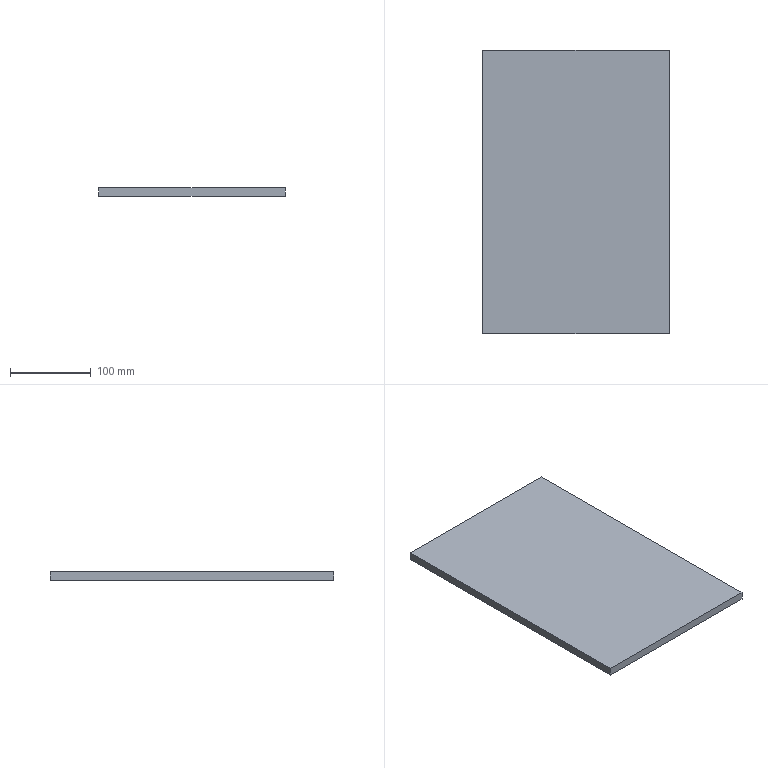Component | SolidWorks | ElectricalCabinetPanel-2 | 1 solid | 6 faces | box 230 x 350 x 10 mm | volume 805000 mm3 | plane 6
build123d program:
from build123d import *

# Parameters (mm, degrees)
SKETCH1_W           = 350
SKETCH1_H           = 230
BOSS_EXTRUDE1_DEPTH = 10


with BuildPart() as part:
    # Sketch1 → Boss-Extrude1 (new body)
    with BuildSketch(Plane.XY):
        with Locations((-175, -115)):
            Rectangle(SKETCH1_W, SKETCH1_H)
    extrude(amount=BOSS_EXTRUDE1_DEPTH)


solid = part.part

# Placed as in the assembly
solid = solid.moved(Location((-920, 370, 90), (0, 0, 90)))
STEP:
#1=CARTESIAN_POINT('',(-27.165,14.567,3.543));
#2=VERTEX_POINT('',#1);
#3=CARTESIAN_POINT('',(-36.22,14.567,3.543));
#4=VERTEX_POINT('',#3);
#5=CARTESIAN_POINT('',(-36.22,14.567,3.543));
#6=DIRECTION('',(-1.,0.,0.));
#7=VECTOR('',#6,39.37);
#8=LINE('',#5,#7);
#9=EDGE_CURVE('',#2,#4,#8,.T.);
#10=ORIENTED_EDGE('',*,*,#9,.T.);
#11=CARTESIAN_POINT('',(-36.22,14.567,3.937));
#12=VERTEX_POINT('',#11);
#13=CARTESIAN_POINT('',(-36.22,14.567,3.937));
#14=DIRECTION('',(0.,0.,-1.));
#15=VECTOR('',#14,39.37);
#16=LINE('',#13,#15);
#17=EDGE_CURVE('',#12,#4,#16,.T.);
#18=ORIENTED_EDGE('',*,*,#17,.F.);
#19=CARTESIAN_POINT('',(-27.165,14.567,3.937));
#20=VERTEX_POINT('',#19);
#21=CARTESIAN_POINT('',(-36.22,14.567,3.937));
#22=DIRECTION('',(-1.,0.,0.));
#23=VECTOR('',#22,39.37);
#24=LINE('',#21,#23);
#25=EDGE_CURVE('',#20,#12,#24,.T.);
#26=ORIENTED_EDGE('',*,*,#25,.F.);
#27=CARTESIAN_POINT('',(-27.165,14.567,3.937));
#28=DIRECTION('',(0.,0.,-1.));
#29=VECTOR('',#28,39.37);
#30=LINE('',#27,#29);
#31=EDGE_CURVE('',#20,#2,#30,.T.);
#32=ORIENTED_EDGE('',*,*,#31,.T.);
#33=EDGE_LOOP('',(#10,#18,#26,#32));
#34=FACE_OUTER_BOUND('',#33,.T.);
#35=CARTESIAN_POINT('',(-36.22,14.567,3.937));
#36=DIRECTION('',(0.,-1.,0.));
#37=DIRECTION('',(0.,0.,-1.));
#38=AXIS2_PLACEMENT_3D('',#35,#36,#37);
#39=PLANE('',#38);
#40=ADVANCED_FACE('',(#34),#39,.F.);
#41=CARTESIAN_POINT('',(-36.22,0.7874,3.543));
#42=VERTEX_POINT('',#41);
#43=CARTESIAN_POINT('',(-36.22,14.567,3.543));
#44=DIRECTION('',(0.,-1.,0.));
#45=VECTOR('',#44,39.37);
#46=LINE('',#43,#45);
#47=EDGE_CURVE('',#4,#42,#46,.T.);
#48=ORIENTED_EDGE('',*,*,#47,.T.);
#49=CARTESIAN_POINT('',(-36.22,0.7874,3.937));
#50=VERTEX_POINT('',#49);
#51=CARTESIAN_POINT('',(-36.22,0.7874,3.937));
#52=DIRECTION('',(0.,0.,-1.));
#53=VECTOR('',#52,39.37);
#54=LINE('',#51,#53);
#55=EDGE_CURVE('',#50,#42,#54,.T.);
#56=ORIENTED_EDGE('',*,*,#55,.F.);
#57=CARTESIAN_POINT('',(-36.22,14.567,3.937));
#58=DIRECTION('',(0.,-1.,0.));
#59=VECTOR('',#58,39.37);
#60=LINE('',#57,#59);
#61=EDGE_CURVE('',#12,#50,#60,.T.);
#62=ORIENTED_EDGE('',*,*,#61,.F.);
#63=ORIENTED_EDGE('',*,*,#17,.T.);
#64=EDGE_LOOP('',(#48,#56,#62,#63));
#65=FACE_OUTER_BOUND('',#64,.T.);
#66=CARTESIAN_POINT('',(-36.22,14.567,3.937));
#67=DIRECTION('',(1.,0.,0.));
#68=DIRECTION('',(0.,0.,1.));
#69=AXIS2_PLACEMENT_3D('',#66,#67,#68);
#70=PLANE('',#69);
#71=ADVANCED_FACE('',(#65),#70,.F.);
#72=CARTESIAN_POINT('',(-27.165,0.7874,3.543));
#73=VERTEX_POINT('',#72);
#74=CARTESIAN_POINT('',(-36.22,0.7874,3.543));
#75=DIRECTION('',(1.,0.,0.));
#76=VECTOR('',#75,39.37);
#77=LINE('',#74,#76);
#78=EDGE_CURVE('',#42,#73,#77,.T.);
#79=ORIENTED_EDGE('',*,*,#78,.T.);
#80=CARTESIAN_POINT('',(-27.165,0.7874,3.937));
#81=VERTEX_POINT('',#80);
#82=CARTESIAN_POINT('',(-27.165,0.7874,3.937));
#83=DIRECTION('',(0.,0.,-1.));
#84=VECTOR('',#83,39.37);
#85=LINE('',#82,#84);
#86=EDGE_CURVE('',#81,#73,#85,.T.);
#87=ORIENTED_EDGE('',*,*,#86,.F.);
#88=CARTESIAN_POINT('',(-36.22,0.7874,3.937));
#89=DIRECTION('',(1.,0.,0.));
#90=VECTOR('',#89,39.37);
#91=LINE('',#88,#90);
#92=EDGE_CURVE('',#50,#81,#91,.T.);
#93=ORIENTED_EDGE('',*,*,#92,.F.);
#94=ORIENTED_EDGE('',*,*,#55,.T.);
#95=EDGE_LOOP('',(#79,#87,#93,#94));
#96=FACE_OUTER_BOUND('',#95,.T.);
#97=CARTESIAN_POINT('',(-36.22,0.7874,3.937));
#98=DIRECTION('',(0.,1.,0.));
#99=DIRECTION('',(0.,0.,1.));
#100=AXIS2_PLACEMENT_3D('',#97,#98,#99);
#101=PLANE('',#100);
#102=ADVANCED_FACE('',(#96),#101,.F.);
#103=CARTESIAN_POINT('',(-27.165,14.567,3.543));
#104=DIRECTION('',(0.,1.,0.));
#105=VECTOR('',#104,39.37);
#106=LINE('',#103,#105);
#107=EDGE_CURVE('',#73,#2,#106,.T.);
#108=ORIENTED_EDGE('',*,*,#107,.T.);
#109=ORIENTED_EDGE('',*,*,#31,.F.);
#110=CARTESIAN_POINT('',(-27.165,14.567,3.937));
#111=DIRECTION('',(0.,1.,0.));
#112=VECTOR('',#111,39.37);
#113=LINE('',#110,#112);
#114=EDGE_CURVE('',#81,#20,#113,.T.);
#115=ORIENTED_EDGE('',*,*,#114,.F.);
#116=ORIENTED_EDGE('',*,*,#86,.T.);
#117=EDGE_LOOP('',(#108,#109,#115,#116));
#118=FACE_OUTER_BOUND('',#117,.T.);
#119=CARTESIAN_POINT('',(-27.165,14.567,3.937));
#120=DIRECTION('',(-1.,0.,0.));
#121=DIRECTION('',(0.,0.,-1.));
#122=AXIS2_PLACEMENT_3D('',#119,#120,#121);
#123=PLANE('',#122);
#124=ADVANCED_FACE('',(#118),#123,.F.);
#125=ORIENTED_EDGE('',*,*,#25,.T.);
#126=ORIENTED_EDGE('',*,*,#61,.T.);
#127=ORIENTED_EDGE('',*,*,#92,.T.);
#128=ORIENTED_EDGE('',*,*,#114,.T.);
#129=EDGE_LOOP('',(#125,#126,#127,#128));
#130=FACE_OUTER_BOUND('',#129,.T.);
#131=CARTESIAN_POINT('',(-27.165,0.7874,3.937));
#132=DIRECTION('',(0.,0.,-1.));
#133=DIRECTION('',(0.,1.,0.));
#134=AXIS2_PLACEMENT_3D('',#131,#132,#133);
#135=PLANE('',#134);
#136=ADVANCED_FACE('',(#130),#135,.F.);
#137=ORIENTED_EDGE('',*,*,#9,.F.);
#138=ORIENTED_EDGE('',*,*,#107,.F.);
#139=ORIENTED_EDGE('',*,*,#78,.F.);
#140=ORIENTED_EDGE('',*,*,#47,.F.);
#141=EDGE_LOOP('',(#137,#138,#139,#140));
#142=FACE_OUTER_BOUND('',#141,.T.);
#143=CARTESIAN_POINT('',(-27.165,0.7874,3.543));
#144=DIRECTION('',(0.,0.,-1.));
#145=DIRECTION('',(0.,1.,0.));
#146=AXIS2_PLACEMENT_3D('',#143,#144,#145);
#147=PLANE('',#146);
#148=ADVANCED_FACE('',(#142),#147,.T.);
#149=CLOSED_SHELL('',(#40,#71,#102,#124,#136,#148));
#150=MANIFOLD_SOLID_BREP('',#149);
#151=CARTESIAN_POINT('',(0.,0.,0.));
#152=DIRECTION('',(0.,0.,1.));
#153=DIRECTION('',(1.,0.,0.));
#154=AXIS2_PLACEMENT_3D('',#151,#152,#153);
#155=(LENGTH_UNIT()NAMED_UNIT(*)SI_UNIT($,.METRE.));
#156=LENGTH_MEASURE_WITH_UNIT(LENGTH_MEASURE(0.0254),#155);
#157=DIMENSIONAL_EXPONENTS(1.,0.,0.,0.,0.,0.,0.);
#158=(CONVERSION_BASED_UNIT('',#156)LENGTH_UNIT()NAMED_UNIT(#157));
#159=UNCERTAINTY_MEASURE_WITH_UNIT(LENGTH_MEASURE(0.00001),#158,'','');
#160=(NAMED_UNIT(*)PLANE_ANGLE_UNIT()SI_UNIT($,.RADIAN.));
#161=(NAMED_UNIT(*)SI_UNIT($,.STERADIAN.)SOLID_ANGLE_UNIT());
#162=(GEOMETRIC_REPRESENTATION_CONTEXT(3)GLOBAL_UNCERTAINTY_ASSIGNED_CONTEXT((#159))GLOBAL_UNIT_ASSIGNED_CONTEXT((#158,#160,#161))REPRESENTATION_CONTEXT('',''));
#163=ADVANCED_BREP_SHAPE_REPRESENTATION('',(#150,#154),#162);
#164=COLOUR_RGB('',0.7922,0.8196,0.9333);
#165=FILL_AREA_STYLE_COLOUR('',#164);
#166=FILL_AREA_STYLE('',(#165));
#167=SURFACE_STYLE_FILL_AREA(#166);
#168=SURFACE_SIDE_STYLE('',(#167));
#169=SURFACE_STYLE_USAGE(.BOTH.,#168);
#170=PRESENTATION_STYLE_ASSIGNMENT((#169));
#171=STYLED_ITEM('',(#170),#150);
#172=PRESENTATION_LAYER_ASSIGNMENT('','',(#171));
#173=(LENGTH_UNIT()NAMED_UNIT(*)SI_UNIT($,.METRE.));
#174=LENGTH_MEASURE_WITH_UNIT(LENGTH_MEASURE(0.0254),#173);
#175=DIMENSIONAL_EXPONENTS(1.,0.,0.,0.,0.,0.,0.);
#176=(CONVERSION_BASED_UNIT('',#174)LENGTH_UNIT()NAMED_UNIT(#175));
#177=UNCERTAINTY_MEASURE_WITH_UNIT(LENGTH_MEASURE(0.00001),#176,'','');
#178=(NAMED_UNIT(*)PLANE_ANGLE_UNIT()SI_UNIT($,.RADIAN.));
#179=(NAMED_UNIT(*)SI_UNIT($,.STERADIAN.)SOLID_ANGLE_UNIT());
#180=(GEOMETRIC_REPRESENTATION_CONTEXT(3)GLOBAL_UNCERTAINTY_ASSIGNED_CONTEXT((#177))GLOBAL_UNIT_ASSIGNED_CONTEXT((#176,#178,#179))REPRESENTATION_CONTEXT('',''));
#181=MECHANICAL_DESIGN_GEOMETRIC_PRESENTATION_REPRESENTATION('',(#171),#180);